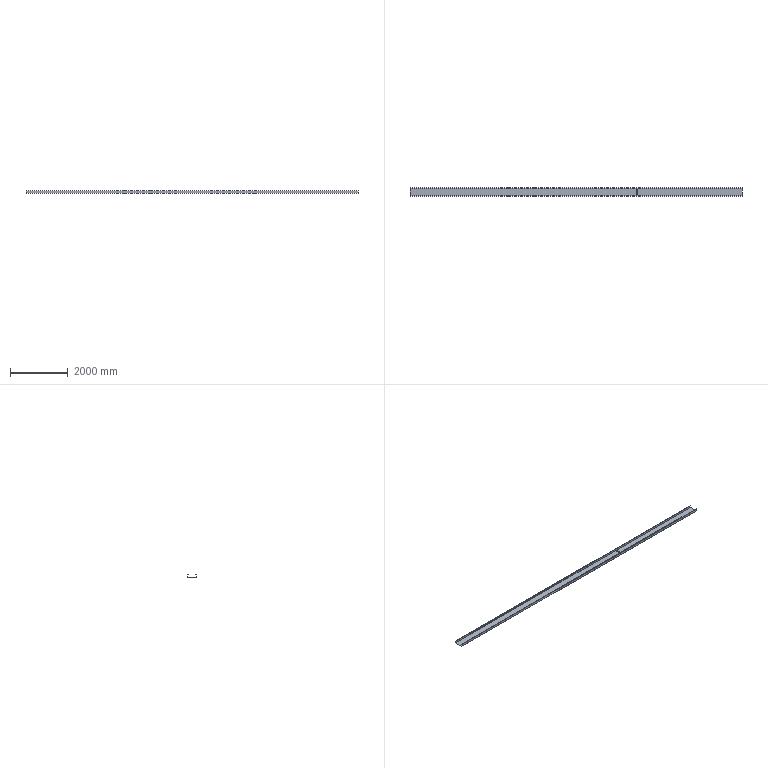Component | NX | DBLIANJIE | 1 solid | 18 faces | volume 16747440 mm3 | plane 18